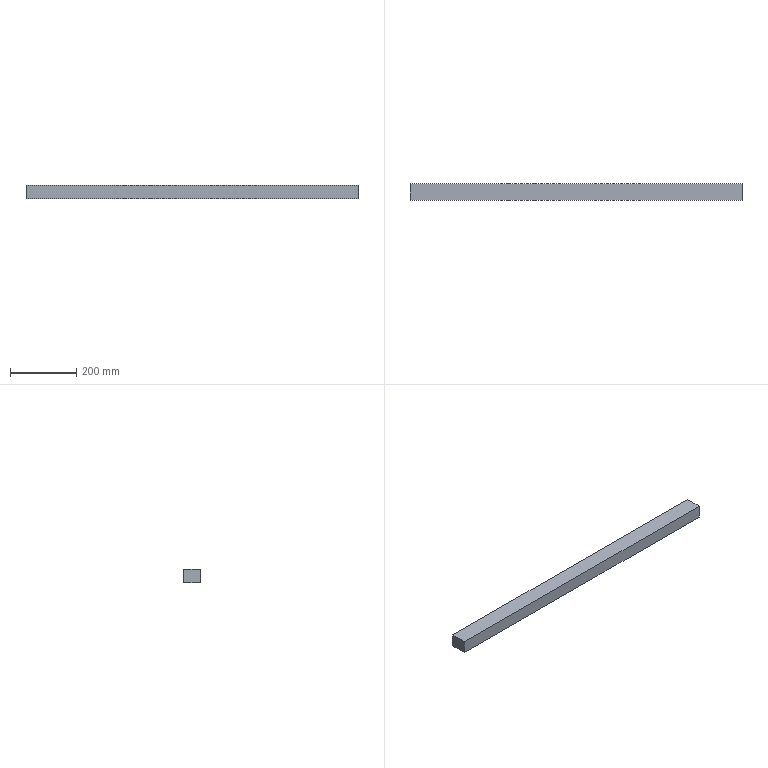Component | SolidWorks | OuterRod-1 | 1 solid | 6 faces | box 1000 x 50 x 40 mm | volume 2000000 mm3 | plane 6
build123d program:
from build123d import *

# Parameters (mm, degrees)
SKETCH1_W           = 1000
SKETCH1_H           = 40
BOSS_EXTRUDE1_DEPTH = 50


with BuildPart() as part:
    # Sketch1 → Boss-Extrude1 (new body)
    with BuildSketch(Plane.XY):
        with Locations((-13.518, 182.763)):
            Rectangle(SKETCH1_W, SKETCH1_H)
    extrude(amount=BOSS_EXTRUDE1_DEPTH)


solid = part.part

# Placed as in the assembly
solid = solid.moved(Location((13.518, 500, -365.526), (90, 0, 0)))
STEP:
#1=COLOUR_RGB('',0.7922,0.8196,0.9333);
#2=FILL_AREA_STYLE_COLOUR('',#1);
#3=FILL_AREA_STYLE('',(#2));
#4=SURFACE_STYLE_FILL_AREA(#3);
#5=SURFACE_SIDE_STYLE('',(#4));
#6=SURFACE_STYLE_USAGE(.BOTH.,#5);
#7=PRESENTATION_STYLE_ASSIGNMENT((#6));
#8=CARTESIAN_POINT('',(-19.685,17.717,-7.983));
#9=VERTEX_POINT('',#8);
#10=CARTESIAN_POINT('',(-19.685,17.717,-6.408));
#11=VERTEX_POINT('',#10);
#12=CARTESIAN_POINT('',(-19.685,17.717,-6.408));
#13=DIRECTION('',(0.,0.,1.));
#14=VECTOR('',#13,39.37);
#15=LINE('',#12,#14);
#16=EDGE_CURVE('',#9,#11,#15,.T.);
#17=ORIENTED_EDGE('',*,*,#16,.T.);
#18=CARTESIAN_POINT('',(-19.685,19.685,-6.408));
#19=VERTEX_POINT('',#18);
#20=CARTESIAN_POINT('',(-19.685,19.685,-6.408));
#21=DIRECTION('',(0.,-1.,0.));
#22=VECTOR('',#21,39.37);
#23=LINE('',#20,#22);
#24=EDGE_CURVE('',#19,#11,#23,.T.);
#25=ORIENTED_EDGE('',*,*,#24,.F.);
#26=CARTESIAN_POINT('',(-19.685,19.685,-7.983));
#27=VERTEX_POINT('',#26);
#28=CARTESIAN_POINT('',(-19.685,19.685,-6.408));
#29=DIRECTION('',(0.,0.,1.));
#30=VECTOR('',#29,39.37);
#31=LINE('',#28,#30);
#32=EDGE_CURVE('',#27,#19,#31,.T.);
#33=ORIENTED_EDGE('',*,*,#32,.F.);
#34=CARTESIAN_POINT('',(-19.685,19.685,-7.983));
#35=DIRECTION('',(0.,-1.,0.));
#36=VECTOR('',#35,39.37);
#37=LINE('',#34,#36);
#38=EDGE_CURVE('',#27,#9,#37,.T.);
#39=ORIENTED_EDGE('',*,*,#38,.T.);
#40=EDGE_LOOP('',(#17,#25,#33,#39));
#41=FACE_OUTER_BOUND('',#40,.T.);
#42=CARTESIAN_POINT('',(-19.685,19.685,-6.408));
#43=DIRECTION('',(1.,0.,0.));
#44=DIRECTION('',(0.,-1.,0.));
#45=AXIS2_PLACEMENT_3D('',#42,#43,#44);
#46=PLANE('',#45);
#47=ADVANCED_FACE('',(#41),#46,.F.);
#48=CARTESIAN_POINT('',(19.685,17.717,-6.408));
#49=VERTEX_POINT('',#48);
#50=CARTESIAN_POINT('',(-19.685,17.717,-6.408));
#51=DIRECTION('',(1.,0.,0.));
#52=VECTOR('',#51,39.37);
#53=LINE('',#50,#52);
#54=EDGE_CURVE('',#11,#49,#53,.T.);
#55=ORIENTED_EDGE('',*,*,#54,.T.);
#56=CARTESIAN_POINT('',(19.685,19.685,-6.408));
#57=VERTEX_POINT('',#56);
#58=CARTESIAN_POINT('',(19.685,19.685,-6.408));
#59=DIRECTION('',(0.,-1.,0.));
#60=VECTOR('',#59,39.37);
#61=LINE('',#58,#60);
#62=EDGE_CURVE('',#57,#49,#61,.T.);
#63=ORIENTED_EDGE('',*,*,#62,.F.);
#64=CARTESIAN_POINT('',(-19.685,19.685,-6.408));
#65=DIRECTION('',(1.,0.,0.));
#66=VECTOR('',#65,39.37);
#67=LINE('',#64,#66);
#68=EDGE_CURVE('',#19,#57,#67,.T.);
#69=ORIENTED_EDGE('',*,*,#68,.F.);
#70=ORIENTED_EDGE('',*,*,#24,.T.);
#71=EDGE_LOOP('',(#55,#63,#69,#70));
#72=FACE_OUTER_BOUND('',#71,.T.);
#73=CARTESIAN_POINT('',(-19.685,19.685,-6.408));
#74=DIRECTION('',(0.,0.,-1.));
#75=DIRECTION('',(0.,1.,0.));
#76=AXIS2_PLACEMENT_3D('',#73,#74,#75);
#77=PLANE('',#76);
#78=ADVANCED_FACE('',(#72),#77,.F.);
#79=CARTESIAN_POINT('',(19.685,17.717,-7.983));
#80=VERTEX_POINT('',#79);
#81=CARTESIAN_POINT('',(19.685,17.717,-6.408));
#82=DIRECTION('',(0.,0.,-1.));
#83=VECTOR('',#82,39.37);
#84=LINE('',#81,#83);
#85=EDGE_CURVE('',#49,#80,#84,.T.);
#86=ORIENTED_EDGE('',*,*,#85,.T.);
#87=CARTESIAN_POINT('',(19.685,19.685,-7.983));
#88=VERTEX_POINT('',#87);
#89=CARTESIAN_POINT('',(19.685,19.685,-7.983));
#90=DIRECTION('',(0.,-1.,0.));
#91=VECTOR('',#90,39.37);
#92=LINE('',#89,#91);
#93=EDGE_CURVE('',#88,#80,#92,.T.);
#94=ORIENTED_EDGE('',*,*,#93,.F.);
#95=CARTESIAN_POINT('',(19.685,19.685,-6.408));
#96=DIRECTION('',(0.,0.,-1.));
#97=VECTOR('',#96,39.37);
#98=LINE('',#95,#97);
#99=EDGE_CURVE('',#57,#88,#98,.T.);
#100=ORIENTED_EDGE('',*,*,#99,.F.);
#101=ORIENTED_EDGE('',*,*,#62,.T.);
#102=EDGE_LOOP('',(#86,#94,#100,#101));
#103=FACE_OUTER_BOUND('',#102,.T.);
#104=CARTESIAN_POINT('',(19.685,19.685,-6.408));
#105=DIRECTION('',(-1.,0.,0.));
#106=DIRECTION('',(0.,1.,0.));
#107=AXIS2_PLACEMENT_3D('',#104,#105,#106);
#108=PLANE('',#107);
#109=ADVANCED_FACE('',(#103),#108,.F.);
#110=CARTESIAN_POINT('',(-19.685,17.717,-7.983));
#111=DIRECTION('',(-1.,0.,-0.));
#112=VECTOR('',#111,39.37);
#113=LINE('',#110,#112);
#114=EDGE_CURVE('',#80,#9,#113,.T.);
#115=ORIENTED_EDGE('',*,*,#114,.T.);
#116=ORIENTED_EDGE('',*,*,#38,.F.);
#117=CARTESIAN_POINT('',(-19.685,19.685,-7.983));
#118=DIRECTION('',(-1.,0.,-0.));
#119=VECTOR('',#118,39.37);
#120=LINE('',#117,#119);
#121=EDGE_CURVE('',#88,#27,#120,.T.);
#122=ORIENTED_EDGE('',*,*,#121,.F.);
#123=ORIENTED_EDGE('',*,*,#93,.T.);
#124=EDGE_LOOP('',(#115,#116,#122,#123));
#125=FACE_OUTER_BOUND('',#124,.T.);
#126=CARTESIAN_POINT('',(-19.685,19.685,-7.983));
#127=DIRECTION('',(-0.,0.,1.));
#128=DIRECTION('',(1.,0.,0.));
#129=AXIS2_PLACEMENT_3D('',#126,#127,#128);
#130=PLANE('',#129);
#131=ADVANCED_FACE('',(#125),#130,.F.);
#132=ORIENTED_EDGE('',*,*,#32,.T.);
#133=ORIENTED_EDGE('',*,*,#68,.T.);
#134=ORIENTED_EDGE('',*,*,#99,.T.);
#135=ORIENTED_EDGE('',*,*,#121,.T.);
#136=EDGE_LOOP('',(#132,#133,#134,#135));
#137=FACE_OUTER_BOUND('',#136,.T.);
#138=CARTESIAN_POINT('',(0.5322,19.685,0.));
#139=DIRECTION('',(0.,-1.,0.));
#140=DIRECTION('',(-1.,0.,0.));
#141=AXIS2_PLACEMENT_3D('',#138,#139,#140);
#142=PLANE('',#141);
#143=ADVANCED_FACE('',(#137),#142,.F.);
#144=ORIENTED_EDGE('',*,*,#16,.F.);
#145=ORIENTED_EDGE('',*,*,#114,.F.);
#146=ORIENTED_EDGE('',*,*,#85,.F.);
#147=ORIENTED_EDGE('',*,*,#54,.F.);
#148=EDGE_LOOP('',(#144,#145,#146,#147));
#149=FACE_OUTER_BOUND('',#148,.T.);
#150=CARTESIAN_POINT('',(0.5322,17.717,0.));
#151=DIRECTION('',(0.,-1.,0.));
#152=DIRECTION('',(-1.,0.,0.));
#153=AXIS2_PLACEMENT_3D('',#150,#151,#152);
#154=PLANE('',#153);
#155=ADVANCED_FACE('',(#149),#154,.T.);
#156=CLOSED_SHELL('',(#47,#78,#109,#131,#143,#155));
#157=MANIFOLD_SOLID_BREP('',#156);
#158=STYLED_ITEM('',(#7),#157);
#159=PRESENTATION_LAYER_ASSIGNMENT('','',(#158));
#160=(LENGTH_UNIT()NAMED_UNIT(*)SI_UNIT($,.METRE.));
#161=LENGTH_MEASURE_WITH_UNIT(LENGTH_MEASURE(0.0254),#160);
#162=DIMENSIONAL_EXPONENTS(1.,0.,0.,0.,0.,0.,0.);
#163=(CONVERSION_BASED_UNIT('',#161)LENGTH_UNIT()NAMED_UNIT(#162));
#164=UNCERTAINTY_MEASURE_WITH_UNIT(LENGTH_MEASURE(0.00001),#163,'','');
#165=(NAMED_UNIT(*)PLANE_ANGLE_UNIT()SI_UNIT($,.RADIAN.));
#166=(NAMED_UNIT(*)SI_UNIT($,.STERADIAN.)SOLID_ANGLE_UNIT());
#167=(GEOMETRIC_REPRESENTATION_CONTEXT(3)GLOBAL_UNCERTAINTY_ASSIGNED_CONTEXT((#164))GLOBAL_UNIT_ASSIGNED_CONTEXT((#163,#165,#166))REPRESENTATION_CONTEXT('',''));
#168=MECHANICAL_DESIGN_GEOMETRIC_PRESENTATION_REPRESENTATION('',(#158),#167);
#169=CARTESIAN_POINT('',(0.,0.,0.));
#170=DIRECTION('',(0.,0.,1.));
#171=DIRECTION('',(1.,0.,0.));
#172=AXIS2_PLACEMENT_3D('',#169,#170,#171);
#173=(LENGTH_UNIT()NAMED_UNIT(*)SI_UNIT($,.METRE.));
#174=LENGTH_MEASURE_WITH_UNIT(LENGTH_MEASURE(0.0254),#173);
#175=DIMENSIONAL_EXPONENTS(1.,0.,0.,0.,0.,0.,0.);
#176=(CONVERSION_BASED_UNIT('',#174)LENGTH_UNIT()NAMED_UNIT(#175));
#177=UNCERTAINTY_MEASURE_WITH_UNIT(LENGTH_MEASURE(0.00001),#176,'','');
#178=(NAMED_UNIT(*)PLANE_ANGLE_UNIT()SI_UNIT($,.RADIAN.));
#179=(NAMED_UNIT(*)SI_UNIT($,.STERADIAN.)SOLID_ANGLE_UNIT());
#180=(GEOMETRIC_REPRESENTATION_CONTEXT(3)GLOBAL_UNCERTAINTY_ASSIGNED_CONTEXT((#177))GLOBAL_UNIT_ASSIGNED_CONTEXT((#176,#178,#179))REPRESENTATION_CONTEXT('',''));
#181=ADVANCED_BREP_SHAPE_REPRESENTATION('',(#157,#172),#180);